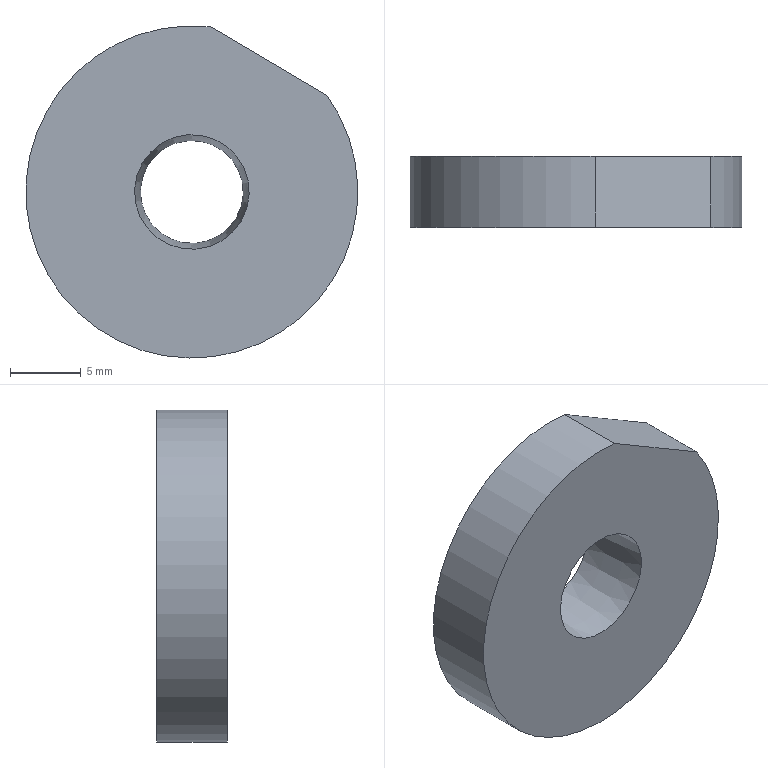Component | NX | CAM | 1 solid | 5 faces | box 23.4 x 5 x 23.4 mm | volume 1887 mm3 | plane 3 | cylinder 1 | cone 1 | commonest cylinder face diameters 23.4 x1
STEP:
#1=CARTESIAN_POINT('',(0.,0.,0.));
#2=DIRECTION('',(0.,0.,1.));
#3=DIRECTION('',(1.,0.,0.));
#4=AXIS2_PLACEMENT_3D('',#1,#2,#3);
#5=CARTESIAN_POINT('',(1.355,39.8,54.921));
#6=VERTEX_POINT('',#5);
#7=CARTESIAN_POINT('',(9.51,39.8,50.116));
#8=VERTEX_POINT('',#7);
#9=CARTESIAN_POINT('',(0.0005589,39.8,43.3));
#10=DIRECTION('',(0.,-1.,0.));
#11=DIRECTION('',(-0.8615,0.,0.5077));
#12=AXIS2_PLACEMENT_3D('',#9,#10,#11);
#13=CIRCLE('',#12,11.7);
#14=CARTESIAN_POINT('',(0.0005589,44.8,43.3));
#15=DIRECTION('',(0.,-1.,0.));
#16=DIRECTION('',(0.8615,0.,-0.5077));
#17=AXIS2_PLACEMENT_3D('',#14,#15,#16);
#18=CYLINDRICAL_SURFACE('',#17,11.7);
#19=CARTESIAN_POINT('',(-3.142,5.));
#20=DIRECTION('',(1.,0.));
#21=VECTOR('',#20,1.);
#22=LINE('',#19,#21);
#23=(GEOMETRIC_REPRESENTATION_CONTEXT(2)PARAMETRIC_REPRESENTATION_CONTEXT()REPRESENTATION_CONTEXT('',''));
#24=DEFINITIONAL_REPRESENTATION('',(#22),#23);
#25=PCURVE('',#18,#24);
#26=CARTESIAN_POINT('',(0.0005589,39.8,43.3));
#27=DIRECTION('',(0.,-1.,0.));
#28=DIRECTION('',(0.8615,0.,-0.5077));
#29=AXIS2_PLACEMENT_3D('',#26,#27,#28);
#30=PLANE('',#29);
#31=CARTESIAN_POINT('',(0.,0.));
#32=DIRECTION('',(-1.,0.));
#33=AXIS2_PLACEMENT_2D('',#31,#32);
#34=CIRCLE('',#33,11.7);
#35=(GEOMETRIC_REPRESENTATION_CONTEXT(2)PARAMETRIC_REPRESENTATION_CONTEXT()REPRESENTATION_CONTEXT('',''));
#36=DEFINITIONAL_REPRESENTATION('',(#34),#35);
#37=PCURVE('',#30,#36);
#38=SURFACE_CURVE('',#13,(#25,#37),.PCURVE_S1.);
#39=EDGE_CURVE('',#6,#8,#38,.T.);
#40=ORIENTED_EDGE('',*,*,#39,.F.);
#41=CARTESIAN_POINT('',(1.355,44.8,54.921));
#42=VERTEX_POINT('',#41);
#43=CARTESIAN_POINT('',(1.355,44.8,54.921));
#44=DIRECTION('',(0.,1.,0.));
#45=VECTOR('',#44,1.);
#46=LINE('',#43,#45);
#47=CARTESIAN_POINT('',(1.987,0.));
#48=DIRECTION('',(0.,-1.));
#49=VECTOR('',#48,1.);
#50=LINE('',#47,#49);
#51=(GEOMETRIC_REPRESENTATION_CONTEXT(2)PARAMETRIC_REPRESENTATION_CONTEXT()REPRESENTATION_CONTEXT('',''));
#52=DEFINITIONAL_REPRESENTATION('',(#50),#51);
#53=PCURVE('',#18,#52);
#54=CARTESIAN_POINT('',(9.51,44.8,50.116));
#55=DIRECTION('',(0.5077,0.,0.8615));
#56=DIRECTION('',(0.,1.,0.));
#57=AXIS2_PLACEMENT_3D('',#54,#55,#56);
#58=PLANE('',#57);
#59=CARTESIAN_POINT('',(0.,9.466));
#60=DIRECTION('',(1.,0.));
#61=VECTOR('',#60,1.);
#62=LINE('',#59,#61);
#63=(GEOMETRIC_REPRESENTATION_CONTEXT(2)PARAMETRIC_REPRESENTATION_CONTEXT()REPRESENTATION_CONTEXT('',''));
#64=DEFINITIONAL_REPRESENTATION('',(#62),#63);
#65=PCURVE('',#58,#64);
#66=SURFACE_CURVE('',#46,(#53,#65),.PCURVE_S1.);
#67=EDGE_CURVE('',#6,#42,#66,.T.);
#68=ORIENTED_EDGE('',*,*,#67,.T.);
#69=CARTESIAN_POINT('',(9.51,44.8,50.116));
#70=VERTEX_POINT('',#69);
#71=CARTESIAN_POINT('',(0.0005589,44.8,43.3));
#72=DIRECTION('',(0.,-1.,0.));
#73=DIRECTION('',(-0.8615,0.,0.5077));
#74=AXIS2_PLACEMENT_3D('',#71,#72,#73);
#75=CIRCLE('',#74,11.7);
#76=CARTESIAN_POINT('',(-3.142,0.));
#77=DIRECTION('',(1.,0.));
#78=VECTOR('',#77,1.);
#79=LINE('',#76,#78);
#80=(GEOMETRIC_REPRESENTATION_CONTEXT(2)PARAMETRIC_REPRESENTATION_CONTEXT()REPRESENTATION_CONTEXT('',''));
#81=DEFINITIONAL_REPRESENTATION('',(#79),#80);
#82=PCURVE('',#18,#81);
#83=CARTESIAN_POINT('',(0.0005589,44.8,43.3));
#84=DIRECTION('',(0.,-1.,0.));
#85=DIRECTION('',(0.8615,0.,-0.5077));
#86=AXIS2_PLACEMENT_3D('',#83,#84,#85);
#87=PLANE('',#86);
#88=CARTESIAN_POINT('',(0.,0.));
#89=DIRECTION('',(-1.,0.));
#90=AXIS2_PLACEMENT_2D('',#88,#89);
#91=CIRCLE('',#90,11.7);
#92=(GEOMETRIC_REPRESENTATION_CONTEXT(2)PARAMETRIC_REPRESENTATION_CONTEXT()REPRESENTATION_CONTEXT('',''));
#93=DEFINITIONAL_REPRESENTATION('',(#91),#92);
#94=PCURVE('',#87,#93);
#95=SURFACE_CURVE('',#75,(#82,#94),.PCURVE_S1.);
#96=EDGE_CURVE('',#42,#70,#95,.T.);
#97=ORIENTED_EDGE('',*,*,#96,.T.);
#98=CARTESIAN_POINT('',(9.51,44.8,50.116));
#99=DIRECTION('',(0.,-1.,0.));
#100=VECTOR('',#99,1.);
#101=LINE('',#98,#100);
#102=CARTESIAN_POINT('',(7.438,0.));
#103=DIRECTION('',(0.,1.));
#104=VECTOR('',#103,1.);
#105=LINE('',#102,#104);
#106=(GEOMETRIC_REPRESENTATION_CONTEXT(2)PARAMETRIC_REPRESENTATION_CONTEXT()REPRESENTATION_CONTEXT('',''));
#107=DEFINITIONAL_REPRESENTATION('',(#105),#106);
#108=PCURVE('',#18,#107);
#109=CARTESIAN_POINT('',(0.,-0.));
#110=DIRECTION('',(-1.,0.));
#111=VECTOR('',#110,1.);
#112=LINE('',#109,#111);
#113=(GEOMETRIC_REPRESENTATION_CONTEXT(2)PARAMETRIC_REPRESENTATION_CONTEXT()REPRESENTATION_CONTEXT('',''));
#114=DEFINITIONAL_REPRESENTATION('',(#112),#113);
#115=PCURVE('',#58,#114);
#116=SURFACE_CURVE('',#101,(#108,#115),.PCURVE_S1.);
#117=EDGE_CURVE('',#70,#8,#116,.T.);
#118=ORIENTED_EDGE('',*,*,#117,.T.);
#119=EDGE_LOOP('',(#40,#68,#97,#118));
#120=FACE_BOUND('',#119,.T.);
#121=ADVANCED_FACE('',(#120),#18,.T.);
#122=CARTESIAN_POINT('',(9.51,39.8,50.116));
#123=DIRECTION('',(-0.8615,0.,0.5077));
#124=VECTOR('',#123,1.);
#125=LINE('',#122,#124);
#126=CARTESIAN_POINT('',(-5.,0.));
#127=DIRECTION('',(0.,1.));
#128=VECTOR('',#127,1.);
#129=LINE('',#126,#128);
#130=(GEOMETRIC_REPRESENTATION_CONTEXT(2)PARAMETRIC_REPRESENTATION_CONTEXT()REPRESENTATION_CONTEXT('',''));
#131=DEFINITIONAL_REPRESENTATION('',(#129),#130);
#132=PCURVE('',#58,#131);
#133=CARTESIAN_POINT('',(4.733,10.7));
#134=DIRECTION('',(-1.,0.));
#135=VECTOR('',#134,1.);
#136=LINE('',#133,#135);
#137=(GEOMETRIC_REPRESENTATION_CONTEXT(2)PARAMETRIC_REPRESENTATION_CONTEXT()REPRESENTATION_CONTEXT('',''));
#138=DEFINITIONAL_REPRESENTATION('',(#136),#137);
#139=PCURVE('',#30,#138);
#140=SURFACE_CURVE('',#125,(#132,#139),.PCURVE_S1.);
#141=EDGE_CURVE('',#8,#6,#140,.T.);
#142=ORIENTED_EDGE('',*,*,#141,.F.);
#143=ORIENTED_EDGE('',*,*,#117,.F.);
#144=CARTESIAN_POINT('',(9.51,44.8,50.116));
#145=DIRECTION('',(-0.8615,0.,0.5077));
#146=VECTOR('',#145,1.);
#147=LINE('',#144,#146);
#148=CARTESIAN_POINT('',(0.,0.));
#149=DIRECTION('',(0.,1.));
#150=VECTOR('',#149,1.);
#151=LINE('',#148,#150);
#152=(GEOMETRIC_REPRESENTATION_CONTEXT(2)PARAMETRIC_REPRESENTATION_CONTEXT()REPRESENTATION_CONTEXT('',''));
#153=DEFINITIONAL_REPRESENTATION('',(#151),#152);
#154=PCURVE('',#58,#153);
#155=CARTESIAN_POINT('',(4.733,10.7));
#156=DIRECTION('',(-1.,0.));
#157=VECTOR('',#156,1.);
#158=LINE('',#155,#157);
#159=(GEOMETRIC_REPRESENTATION_CONTEXT(2)PARAMETRIC_REPRESENTATION_CONTEXT()REPRESENTATION_CONTEXT('',''));
#160=DEFINITIONAL_REPRESENTATION('',(#158),#159);
#161=PCURVE('',#87,#160);
#162=SURFACE_CURVE('',#147,(#154,#161),.PCURVE_S1.);
#163=EDGE_CURVE('',#70,#42,#162,.T.);
#164=ORIENTED_EDGE('',*,*,#163,.T.);
#165=ORIENTED_EDGE('',*,*,#67,.F.);
#166=EDGE_LOOP('',(#142,#143,#164,#165));
#167=FACE_BOUND('',#166,.T.);
#168=ADVANCED_FACE('',(#167),#58,.T.);
#169=CARTESIAN_POINT('',(-3.123,44.8,45.14));
#170=VERTEX_POINT('',#169);
#171=CARTESIAN_POINT('',(0.0005589,44.8,43.3));
#172=DIRECTION('',(0.,-1.,0.));
#173=DIRECTION('',(-0.8615,0.,0.5077));
#174=AXIS2_PLACEMENT_3D('',#171,#172,#173);
#175=CIRCLE('',#174,3.625);
#176=CARTESIAN_POINT('',(0.,0.));
#177=DIRECTION('',(-1.,-0.));
#178=AXIS2_PLACEMENT_2D('',#176,#177);
#179=CIRCLE('',#178,3.625);
#180=(GEOMETRIC_REPRESENTATION_CONTEXT(2)PARAMETRIC_REPRESENTATION_CONTEXT()REPRESENTATION_CONTEXT('',''));
#181=DEFINITIONAL_REPRESENTATION('',(#179),#180);
#182=PCURVE('',#87,#181);
#183=CARTESIAN_POINT('',(0.0005589,44.8,43.3));
#184=DIRECTION('',(0.,-1.,0.));
#185=DIRECTION('',(-0.8615,0.,0.5077));
#186=AXIS2_PLACEMENT_3D('',#183,#184,#185);
#187=CONICAL_SURFACE('',#186,3.625,0.08314);
#188=CARTESIAN_POINT('',(0.,-0.));
#189=DIRECTION('',(1.,0.));
#190=VECTOR('',#189,1.);
#191=LINE('',#188,#190);
#192=(GEOMETRIC_REPRESENTATION_CONTEXT(2)PARAMETRIC_REPRESENTATION_CONTEXT()REPRESENTATION_CONTEXT('',''));
#193=DEFINITIONAL_REPRESENTATION('',(#191),#192);
#194=PCURVE('',#187,#193);
#195=SURFACE_CURVE('',#175,(#182,#194),.PCURVE_S1.);
#196=EDGE_CURVE('',#170,#170,#195,.T.);
#197=ORIENTED_EDGE('',*,*,#196,.T.);
#198=EDGE_LOOP('',(#197));
#199=FACE_BOUND('',#198,.T.);
#200=ORIENTED_EDGE('',*,*,#96,.F.);
#201=ORIENTED_EDGE('',*,*,#163,.F.);
#202=EDGE_LOOP('',(#200,#201));
#203=FACE_BOUND('',#202,.T.);
#204=ADVANCED_FACE('',(#199,#203),#87,.F.);
#205=CARTESIAN_POINT('',(3.483,39.8,41.248));
#206=VERTEX_POINT('',#205);
#207=CARTESIAN_POINT('',(-3.482,39.8,45.352));
#208=VERTEX_POINT('',#207);
#209=CARTESIAN_POINT('',(0.0005589,39.8,43.3));
#210=DIRECTION('',(0.,-1.,0.));
#211=DIRECTION('',(0.8615,0.,-0.5077));
#212=AXIS2_PLACEMENT_3D('',#209,#210,#211);
#213=CIRCLE('',#212,4.042);
#214=CARTESIAN_POINT('',(0.,0.));
#215=DIRECTION('',(1.,-0.));
#216=AXIS2_PLACEMENT_2D('',#214,#215);
#217=CIRCLE('',#216,4.042);
#218=(GEOMETRIC_REPRESENTATION_CONTEXT(2)PARAMETRIC_REPRESENTATION_CONTEXT()REPRESENTATION_CONTEXT('',''));
#219=DEFINITIONAL_REPRESENTATION('',(#217),#218);
#220=PCURVE('',#30,#219);
#221=CARTESIAN_POINT('',(3.142,5.));
#222=DIRECTION('',(1.,0.));
#223=VECTOR('',#222,1.);
#224=LINE('',#221,#223);
#225=(GEOMETRIC_REPRESENTATION_CONTEXT(2)PARAMETRIC_REPRESENTATION_CONTEXT()REPRESENTATION_CONTEXT('',''));
#226=DEFINITIONAL_REPRESENTATION('',(#224),#225);
#227=PCURVE('',#187,#226);
#228=SURFACE_CURVE('',#213,(#220,#227),.PCURVE_S1.);
#229=EDGE_CURVE('',#206,#208,#228,.T.);
#230=ORIENTED_EDGE('',*,*,#229,.F.);
#231=CARTESIAN_POINT('',(0.0005589,39.8,43.3));
#232=DIRECTION('',(0.,-1.,0.));
#233=DIRECTION('',(0.8615,0.,-0.5077));
#234=AXIS2_PLACEMENT_3D('',#231,#232,#233);
#235=CIRCLE('',#234,4.042);
#236=CARTESIAN_POINT('',(0.,0.));
#237=DIRECTION('',(1.,-0.));
#238=AXIS2_PLACEMENT_2D('',#236,#237);
#239=CIRCLE('',#238,4.042);
#240=(GEOMETRIC_REPRESENTATION_CONTEXT(2)PARAMETRIC_REPRESENTATION_CONTEXT()REPRESENTATION_CONTEXT('',''));
#241=DEFINITIONAL_REPRESENTATION('',(#239),#240);
#242=PCURVE('',#30,#241);
#243=CARTESIAN_POINT('',(-3.142,5.));
#244=DIRECTION('',(1.,0.));
#245=VECTOR('',#244,1.);
#246=LINE('',#243,#245);
#247=(GEOMETRIC_REPRESENTATION_CONTEXT(2)PARAMETRIC_REPRESENTATION_CONTEXT()REPRESENTATION_CONTEXT('',''));
#248=DEFINITIONAL_REPRESENTATION('',(#246),#247);
#249=PCURVE('',#187,#248);
#250=SURFACE_CURVE('',#235,(#242,#249),.PCURVE_S1.);
#251=EDGE_CURVE('',#208,#206,#250,.T.);
#252=ORIENTED_EDGE('',*,*,#251,.F.);
#253=EDGE_LOOP('',(#230,#252));
#254=FACE_BOUND('',#253,.T.);
#255=ORIENTED_EDGE('',*,*,#39,.T.);
#256=ORIENTED_EDGE('',*,*,#141,.T.);
#257=EDGE_LOOP('',(#255,#256));
#258=FACE_BOUND('',#257,.T.);
#259=ADVANCED_FACE('',(#254,#258),#30,.T.);
#260=ORIENTED_EDGE('',*,*,#251,.F.);
#261=CARTESIAN_POINT('',(-3.123,44.8,45.14));
#262=CARTESIAN_POINT('',(-3.482,39.8,45.352));
#263=B_SPLINE_CURVE_WITH_KNOTS('',1,(#261,#262),.UNSPECIFIED.,.F.,.F.,(2,2),(-0.,5.017),.PIECEWISE_BEZIER_KNOTS.);
#264=CARTESIAN_POINT('',(0.,0.));
#265=DIRECTION('',(0.,1.));
#266=VECTOR('',#265,1.);
#267=LINE('',#264,#266);
#268=(GEOMETRIC_REPRESENTATION_CONTEXT(2)PARAMETRIC_REPRESENTATION_CONTEXT()REPRESENTATION_CONTEXT('',''));
#269=DEFINITIONAL_REPRESENTATION('',(#267),#268);
#270=PCURVE('',#187,#269);
#271=CARTESIAN_POINT('',(6.283,0.));
#272=DIRECTION('',(0.,1.));
#273=VECTOR('',#272,1.);
#274=LINE('',#271,#273);
#275=(GEOMETRIC_REPRESENTATION_CONTEXT(2)PARAMETRIC_REPRESENTATION_CONTEXT()REPRESENTATION_CONTEXT('',''));
#276=DEFINITIONAL_REPRESENTATION('',(#274),#275);
#277=PCURVE('',#187,#276);
#278=SEAM_CURVE('',#263,(#270,#277),.PCURVE_S1.);
#279=EDGE_CURVE('',#170,#208,#278,.T.);
#280=ORIENTED_EDGE('',*,*,#279,.F.);
#281=ORIENTED_EDGE('',*,*,#196,.T.);
#282=ORIENTED_EDGE('',*,*,#279,.T.);
#283=ORIENTED_EDGE('',*,*,#229,.F.);
#284=EDGE_LOOP('',(#260,#280,#281,#282,#283));
#285=FACE_BOUND('',#284,.F.);
#286=ADVANCED_FACE('',(#285),#187,.F.);
#287=CLOSED_SHELL('',(#121,#168,#204,#259,#286));
#288=MANIFOLD_SOLID_BREP('',#287);
#289=(LENGTH_UNIT()NAMED_UNIT(*)SI_UNIT(.MILLI.,.METRE.));
#290=UNCERTAINTY_MEASURE_WITH_UNIT(LENGTH_MEASURE(0.000002),#289,'','');
#291=(NAMED_UNIT(*)PLANE_ANGLE_UNIT()SI_UNIT($,.RADIAN.));
#292=(NAMED_UNIT(*)SI_UNIT($,.STERADIAN.)SOLID_ANGLE_UNIT());
#293=(GEOMETRIC_REPRESENTATION_CONTEXT(3)GLOBAL_UNCERTAINTY_ASSIGNED_CONTEXT((#290))GLOBAL_UNIT_ASSIGNED_CONTEXT((#289,#291,#292))REPRESENTATION_CONTEXT('',''));
#294=ADVANCED_BREP_SHAPE_REPRESENTATION('',(#4,#288),#293);